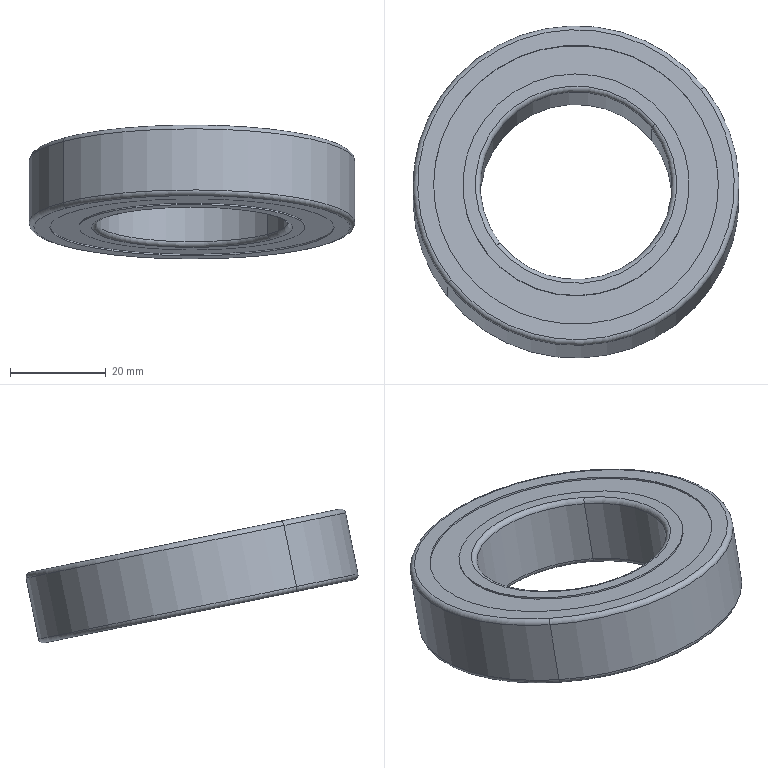Component | SolidWorks | B6008ZZ-2 | 1 solid | 26 faces | box 68 x 69.27 x 27.93 mm | volume 34781 mm3 | cylinder 12 | torus 8 | plane 6 | commonest cylinder face diameters 47.2 x4 59.4 x4 68 x2 40 x2
build123d program:
from build123d import *


with BuildPart() as part:
    # Sketch1 → Revolve1 (revolve)
    with BuildSketch(Plane.XY, mode=Mode.PRIVATE) as revolve1_sk:
        with BuildLine():
            Line((1, 20), (14, 20))
            ThreePointArc((14, 20), (14.707, 20.293), (15, 21))
            Line((15, 21), (15, 23.6))
            Line((15, 23.6), (14.658, 23.6))
            Line((14.658, 23.6), (14.658, 29.7))
            Line((14.658, 29.7), (15, 29.7))
            Line((15, 29.7), (15, 33))
            ThreePointArc((15, 33), (14.707, 33.707), (14, 34))
            Line((14, 34), (1, 34))
            ThreePointArc((1, 34), (0.2929, 33.707), (0, 33))
            Line((0, 33), (0, 29.7))
            Line((0, 29.7), (0.342, 29.7))
            Line((0.342, 29.7), (0.342, 23.6))
            Line((0.342, 23.6), (0, 23.6))
            Line((0, 23.6), (0, 21))
            ThreePointArc((0, 21), (0.2929, 20.293), (1, 20))
        make_face()
    revolve(revolve1_sk.sketch.rotate(Axis((15, 0, 0), (-1, 0, 0)), 270), axis=Axis((15, 0, 0), (-1, 0, 0)))


solid = part.part

# Placed as in the assembly
solid = solid.moved(Location((0, 169.727, 2.1), (78.465, 89.752, 90)))
STEP:
#1=CARTESIAN_POINT('',(-0.733,6.125,0.21));
#2=VERTEX_POINT('',#1);
#3=CARTESIAN_POINT('',(0.733,7.244,-0.01832));
#4=VERTEX_POINT('',#3);
#5=CARTESIAN_POINT('',(-0.,6.685,0.09585));
#6=DIRECTION('',(0.,-0.2,-0.9798));
#7=DIRECTION('',(-0.7889,-0.6021,0.1229));
#8=AXIS2_PLACEMENT_3D('',#5,#6,#7);
#9=CIRCLE('',#8,0.9291);
#10=EDGE_CURVE('',#2,#4,#9,.T.);
#11=ORIENTED_EDGE('',*,*,#10,.T.);
#12=CARTESIAN_POINT('',(0.733,7.242,-0.03152));
#13=VERTEX_POINT('',#12);
#14=CARTESIAN_POINT('',(0.733,7.36,0.5471));
#15=DIRECTION('',(0.,-0.2,-0.9798));
#16=VECTOR('',#15,39.37);
#17=LINE('',#14,#16);
#18=EDGE_CURVE('',#4,#13,#17,.T.);
#19=ORIENTED_EDGE('',*,*,#18,.T.);
#20=CARTESIAN_POINT('',(-0.733,6.123,0.1968));
#21=VERTEX_POINT('',#20);
#22=CARTESIAN_POINT('',(-0.,6.682,0.08266));
#23=DIRECTION('',(0.,-0.2,-0.9798));
#24=DIRECTION('',(-0.7889,-0.6021,0.1229));
#25=AXIS2_PLACEMENT_3D('',#22,#23,#24);
#26=CIRCLE('',#25,0.9291);
#27=EDGE_CURVE('',#21,#13,#26,.T.);
#28=ORIENTED_EDGE('',*,*,#27,.F.);
#29=CARTESIAN_POINT('',(-0.733,6.241,0.7755));
#30=DIRECTION('',(0.,-0.2,-0.9798));
#31=VECTOR('',#30,39.37);
#32=LINE('',#29,#31);
#33=EDGE_CURVE('',#2,#21,#32,.T.);
#34=ORIENTED_EDGE('',*,*,#33,.F.);
#35=EDGE_LOOP('',(#11,#19,#28,#34));
#36=FACE_OUTER_BOUND('',#35,.T.);
#37=CARTESIAN_POINT('',(-0.,6.8,0.6613));
#38=DIRECTION('',(0.,-0.2,-0.9798));
#39=DIRECTION('',(-0.7889,-0.6021,0.1229));
#40=AXIS2_PLACEMENT_3D('',#37,#38,#39);
#41=CYLINDRICAL_SURFACE('',#40,0.9291);
#42=ADVANCED_FACE('',(#36),#41,.T.);
#43=CARTESIAN_POINT('',(0.9224,7.389,-0.04784));
#44=VERTEX_POINT('',#43);
#45=CARTESIAN_POINT('',(-0.9224,5.981,0.2395));
#46=VERTEX_POINT('',#45);
#47=CARTESIAN_POINT('',(-0.,6.685,0.09585));
#48=DIRECTION('',(0.,-0.2,-0.9798));
#49=DIRECTION('',(-0.7889,-0.6021,0.1229));
#50=AXIS2_PLACEMENT_3D('',#47,#48,#49);
#51=CIRCLE('',#50,1.169);
#52=EDGE_CURVE('',#44,#46,#51,.T.);
#53=ORIENTED_EDGE('',*,*,#52,.F.);
#54=CARTESIAN_POINT('',(0.9224,7.386,-0.06103));
#55=VERTEX_POINT('',#54);
#56=CARTESIAN_POINT('',(0.9224,7.504,0.5176));
#57=DIRECTION('',(0.,-0.2,-0.9798));
#58=VECTOR('',#57,39.37);
#59=LINE('',#56,#58);
#60=EDGE_CURVE('',#44,#55,#59,.T.);
#61=ORIENTED_EDGE('',*,*,#60,.T.);
#62=CARTESIAN_POINT('',(-0.9224,5.978,0.2263));
#63=VERTEX_POINT('',#62);
#64=CARTESIAN_POINT('',(-0.,6.682,0.08266));
#65=DIRECTION('',(0.,-0.2,-0.9798));
#66=DIRECTION('',(-0.7889,-0.6021,0.1229));
#67=AXIS2_PLACEMENT_3D('',#64,#65,#66);
#68=CIRCLE('',#67,1.169);
#69=EDGE_CURVE('',#55,#63,#68,.T.);
#70=ORIENTED_EDGE('',*,*,#69,.T.);
#71=CARTESIAN_POINT('',(-0.9224,6.096,0.805));
#72=DIRECTION('',(0.,-0.2,-0.9798));
#73=VECTOR('',#72,39.37);
#74=LINE('',#71,#73);
#75=EDGE_CURVE('',#46,#63,#74,.T.);
#76=ORIENTED_EDGE('',*,*,#75,.F.);
#77=EDGE_LOOP('',(#53,#61,#70,#76));
#78=FACE_OUTER_BOUND('',#77,.T.);
#79=CARTESIAN_POINT('',(-0.,6.8,0.6613));
#80=DIRECTION('',(0.,-0.2,-0.9798));
#81=DIRECTION('',(-0.7889,-0.6021,0.1229));
#82=AXIS2_PLACEMENT_3D('',#79,#80,#81);
#83=CYLINDRICAL_SURFACE('',#82,1.169);
#84=ADVANCED_FACE('',(#78),#83,.F.);
#85=CARTESIAN_POINT('',(-1.056,5.884,0.2857));
#86=VERTEX_POINT('',#85);
#87=CARTESIAN_POINT('',(1.056,7.496,-0.04326));
#88=VERTEX_POINT('',#87);
#89=CARTESIAN_POINT('',(-0.,6.69,0.1212));
#90=DIRECTION('',(0.,-0.2,-0.9798));
#91=DIRECTION('',(-0.7889,-0.6021,0.1229));
#92=AXIS2_PLACEMENT_3D('',#89,#90,#91);
#93=CIRCLE('',#92,1.339);
#94=EDGE_CURVE('',#86,#88,#93,.T.);
#95=ORIENTED_EDGE('',*,*,#94,.T.);
#96=CARTESIAN_POINT('',(1.025,7.464,-0.07699));
#97=VERTEX_POINT('',#96);
#98=CARTESIAN_POINT('',(1.025,7.472,-0.03842));
#99=DIRECTION('',(-0.6145,0.7729,-0.1577));
#100=DIRECTION('',(-0.7827,-0.6223,0.));
#101=AXIS2_PLACEMENT_3D('',#98,#99,#100);
#102=CIRCLE('',#101,0.03937);
#103=EDGE_CURVE('',#88,#97,#102,.T.);
#104=ORIENTED_EDGE('',*,*,#103,.T.);
#105=CARTESIAN_POINT('',(-1.025,5.9,0.2423));
#106=VERTEX_POINT('',#105);
#107=CARTESIAN_POINT('',(-0.,6.682,0.08266));
#108=DIRECTION('',(0.,-0.2,-0.9798));
#109=DIRECTION('',(-0.7889,-0.6021,0.1229));
#110=AXIS2_PLACEMENT_3D('',#107,#108,#109);
#111=CIRCLE('',#110,1.299);
#112=EDGE_CURVE('',#106,#97,#111,.T.);
#113=ORIENTED_EDGE('',*,*,#112,.F.);
#114=CARTESIAN_POINT('',(-1.025,5.908,0.2809));
#115=DIRECTION('',(0.6145,-0.7729,0.1577));
#116=DIRECTION('',(0.7827,0.6223,0.));
#117=AXIS2_PLACEMENT_3D('',#114,#115,#116);
#118=CIRCLE('',#117,0.03937);
#119=EDGE_CURVE('',#86,#106,#118,.T.);
#120=ORIENTED_EDGE('',*,*,#119,.F.);
#121=EDGE_LOOP('',(#95,#104,#113,#120));
#122=FACE_OUTER_BOUND('',#121,.T.);
#123=CARTESIAN_POINT('',(-0.,6.69,0.1212));
#124=DIRECTION('',(0.,-0.2,-0.9798));
#125=DIRECTION('',(-0.7889,-0.6021,0.1229));
#126=AXIS2_PLACEMENT_3D('',#123,#124,#125);
#127=TOROIDAL_SURFACE('',#126,1.299,0.03937);
#128=ADVANCED_FACE('',(#122),#127,.T.);
#129=CARTESIAN_POINT('',(-1.056,5.986,0.7872));
#130=VERTEX_POINT('',#129);
#131=CARTESIAN_POINT('',(1.056,7.598,0.4582));
#132=VERTEX_POINT('',#131);
#133=CARTESIAN_POINT('',(-0.,6.792,0.6227));
#134=DIRECTION('',(0.,-0.2,-0.9798));
#135=DIRECTION('',(-0.7889,-0.6021,0.1229));
#136=AXIS2_PLACEMENT_3D('',#133,#134,#135);
#137=CIRCLE('',#136,1.339);
#138=EDGE_CURVE('',#130,#132,#137,.T.);
#139=ORIENTED_EDGE('',*,*,#138,.T.);
#140=CARTESIAN_POINT('',(1.056,7.606,0.4968));
#141=DIRECTION('',(0.,-0.2,-0.9798));
#142=VECTOR('',#141,39.37);
#143=LINE('',#140,#142);
#144=EDGE_CURVE('',#132,#88,#143,.T.);
#145=ORIENTED_EDGE('',*,*,#144,.T.);
#146=ORIENTED_EDGE('',*,*,#94,.F.);
#147=CARTESIAN_POINT('',(-1.056,5.994,0.8258));
#148=DIRECTION('',(0.,-0.2,-0.9798));
#149=VECTOR('',#148,39.37);
#150=LINE('',#147,#149);
#151=EDGE_CURVE('',#130,#86,#150,.T.);
#152=ORIENTED_EDGE('',*,*,#151,.F.);
#153=EDGE_LOOP('',(#139,#145,#146,#152));
#154=FACE_OUTER_BOUND('',#153,.T.);
#155=CARTESIAN_POINT('',(-0.,6.8,0.6613));
#156=DIRECTION('',(0.,-0.2,-0.9798));
#157=DIRECTION('',(-0.7889,-0.6021,0.1229));
#158=AXIS2_PLACEMENT_3D('',#155,#156,#157);
#159=CYLINDRICAL_SURFACE('',#158,1.339);
#160=ADVANCED_FACE('',(#154),#159,.T.);
#161=CARTESIAN_POINT('',(-1.025,6.018,0.8209));
#162=VERTEX_POINT('',#161);
#163=CARTESIAN_POINT('',(1.025,7.583,0.5016));
#164=VERTEX_POINT('',#163);
#165=CARTESIAN_POINT('',(-0.,6.8,0.6613));
#166=DIRECTION('',(0.,-0.2,-0.9798));
#167=DIRECTION('',(-0.7889,-0.6021,0.1229));
#168=AXIS2_PLACEMENT_3D('',#165,#166,#167);
#169=CIRCLE('',#168,1.299);
#170=EDGE_CURVE('',#162,#164,#169,.T.);
#171=ORIENTED_EDGE('',*,*,#170,.T.);
#172=CARTESIAN_POINT('',(1.025,7.575,0.4631));
#173=DIRECTION('',(-0.6145,0.7729,-0.1577));
#174=DIRECTION('',(-0.7827,-0.6223,0.));
#175=AXIS2_PLACEMENT_3D('',#172,#173,#174);
#176=CIRCLE('',#175,0.03937);
#177=EDGE_CURVE('',#164,#132,#176,.T.);
#178=ORIENTED_EDGE('',*,*,#177,.T.);
#179=ORIENTED_EDGE('',*,*,#138,.F.);
#180=CARTESIAN_POINT('',(-1.025,6.01,0.7824));
#181=DIRECTION('',(0.6145,-0.7729,0.1577));
#182=DIRECTION('',(0.7827,0.6223,0.));
#183=AXIS2_PLACEMENT_3D('',#180,#181,#182);
#184=CIRCLE('',#183,0.03937);
#185=EDGE_CURVE('',#162,#130,#184,.T.);
#186=ORIENTED_EDGE('',*,*,#185,.F.);
#187=EDGE_LOOP('',(#171,#178,#179,#186));
#188=FACE_OUTER_BOUND('',#187,.T.);
#189=CARTESIAN_POINT('',(-0.,6.792,0.6227));
#190=DIRECTION('',(0.,-0.2,-0.9798));
#191=DIRECTION('',(-0.7889,-0.6021,0.1229));
#192=AXIS2_PLACEMENT_3D('',#189,#190,#191);
#193=TOROIDAL_SURFACE('',#192,1.299,0.03937);
#194=ADVANCED_FACE('',(#188),#193,.T.);
#195=CARTESIAN_POINT('',(0.9224,7.504,0.5176));
#196=VERTEX_POINT('',#195);
#197=CARTESIAN_POINT('',(-0.9224,6.096,0.805));
#198=VERTEX_POINT('',#197);
#199=CARTESIAN_POINT('',(-0.,6.8,0.6613));
#200=DIRECTION('',(0.,-0.2,-0.9798));
#201=DIRECTION('',(-0.7889,-0.6021,0.1229));
#202=AXIS2_PLACEMENT_3D('',#199,#200,#201);
#203=CIRCLE('',#202,1.169);
#204=EDGE_CURVE('',#196,#198,#203,.T.);
#205=ORIENTED_EDGE('',*,*,#204,.F.);
#206=CARTESIAN_POINT('',(0.9224,7.502,0.5044));
#207=VERTEX_POINT('',#206);
#208=CARTESIAN_POINT('',(0.9224,7.504,0.5176));
#209=DIRECTION('',(0.,-0.2,-0.9798));
#210=VECTOR('',#209,39.37);
#211=LINE('',#208,#210);
#212=EDGE_CURVE('',#196,#207,#211,.T.);
#213=ORIENTED_EDGE('',*,*,#212,.T.);
#214=CARTESIAN_POINT('',(-0.9224,6.093,0.7918));
#215=VERTEX_POINT('',#214);
#216=CARTESIAN_POINT('',(-0.,6.798,0.6481));
#217=DIRECTION('',(0.,-0.2,-0.9798));
#218=DIRECTION('',(-0.7889,-0.6021,0.1229));
#219=AXIS2_PLACEMENT_3D('',#216,#217,#218);
#220=CIRCLE('',#219,1.169);
#221=EDGE_CURVE('',#207,#215,#220,.T.);
#222=ORIENTED_EDGE('',*,*,#221,.T.);
#223=CARTESIAN_POINT('',(-0.9224,6.096,0.805));
#224=DIRECTION('',(0.,-0.2,-0.9798));
#225=VECTOR('',#224,39.37);
#226=LINE('',#223,#225);
#227=EDGE_CURVE('',#198,#215,#226,.T.);
#228=ORIENTED_EDGE('',*,*,#227,.F.);
#229=EDGE_LOOP('',(#205,#213,#222,#228));
#230=FACE_OUTER_BOUND('',#229,.T.);
#231=CARTESIAN_POINT('',(-0.,6.8,0.6613));
#232=DIRECTION('',(0.,-0.2,-0.9798));
#233=DIRECTION('',(-0.7889,-0.6021,0.1229));
#234=AXIS2_PLACEMENT_3D('',#231,#232,#233);
#235=CYLINDRICAL_SURFACE('',#234,1.169);
#236=ADVANCED_FACE('',(#230),#235,.F.);
#237=CARTESIAN_POINT('',(-0.733,6.241,0.7755));
#238=VERTEX_POINT('',#237);
#239=CARTESIAN_POINT('',(0.733,7.36,0.5471));
#240=VERTEX_POINT('',#239);
#241=CARTESIAN_POINT('',(-0.,6.8,0.6613));
#242=DIRECTION('',(0.,-0.2,-0.9798));
#243=DIRECTION('',(-0.7889,-0.6021,0.1229));
#244=AXIS2_PLACEMENT_3D('',#241,#242,#243);
#245=CIRCLE('',#244,0.9291);
#246=EDGE_CURVE('',#238,#240,#245,.T.);
#247=ORIENTED_EDGE('',*,*,#246,.T.);
#248=CARTESIAN_POINT('',(0.733,7.357,0.5339));
#249=VERTEX_POINT('',#248);
#250=CARTESIAN_POINT('',(0.733,7.36,0.5471));
#251=DIRECTION('',(0.,-0.2,-0.9798));
#252=VECTOR('',#251,39.37);
#253=LINE('',#250,#252);
#254=EDGE_CURVE('',#240,#249,#253,.T.);
#255=ORIENTED_EDGE('',*,*,#254,.T.);
#256=CARTESIAN_POINT('',(-0.733,6.238,0.7623));
#257=VERTEX_POINT('',#256);
#258=CARTESIAN_POINT('',(-0.,6.798,0.6481));
#259=DIRECTION('',(0.,-0.2,-0.9798));
#260=DIRECTION('',(-0.7889,-0.6021,0.1229));
#261=AXIS2_PLACEMENT_3D('',#258,#259,#260);
#262=CIRCLE('',#261,0.9291);
#263=EDGE_CURVE('',#257,#249,#262,.T.);
#264=ORIENTED_EDGE('',*,*,#263,.F.);
#265=CARTESIAN_POINT('',(-0.733,6.241,0.7755));
#266=DIRECTION('',(0.,-0.2,-0.9798));
#267=VECTOR('',#266,39.37);
#268=LINE('',#265,#267);
#269=EDGE_CURVE('',#238,#257,#268,.T.);
#270=ORIENTED_EDGE('',*,*,#269,.F.);
#271=EDGE_LOOP('',(#247,#255,#264,#270));
#272=FACE_OUTER_BOUND('',#271,.T.);
#273=CARTESIAN_POINT('',(-0.,6.8,0.6613));
#274=DIRECTION('',(0.,-0.2,-0.9798));
#275=DIRECTION('',(-0.7889,-0.6021,0.1229));
#276=AXIS2_PLACEMENT_3D('',#273,#274,#275);
#277=CYLINDRICAL_SURFACE('',#276,0.9291);
#278=ADVANCED_FACE('',(#272),#277,.T.);
#279=CARTESIAN_POINT('',(-0.6212,6.318,0.7195));
#280=VERTEX_POINT('',#279);
#281=CARTESIAN_POINT('',(0.6212,7.267,0.526));
#282=VERTEX_POINT('',#281);
#283=CARTESIAN_POINT('',(-0.,6.792,0.6227));
#284=DIRECTION('',(0.,-0.2,-0.9798));
#285=DIRECTION('',(-0.7889,-0.6021,0.1229));
#286=AXIS2_PLACEMENT_3D('',#283,#284,#285);
#287=CIRCLE('',#286,0.7874);
#288=EDGE_CURVE('',#280,#282,#287,.T.);
#289=ORIENTED_EDGE('',*,*,#288,.T.);
#290=CARTESIAN_POINT('',(0.6522,7.298,0.5597));
#291=VERTEX_POINT('',#290);
#292=CARTESIAN_POINT('',(0.6522,7.29,0.5211));
#293=DIRECTION('',(-0.6145,0.7729,-0.1577));
#294=DIRECTION('',(-0.7827,-0.6223,0.));
#295=AXIS2_PLACEMENT_3D('',#292,#293,#294);
#296=CIRCLE('',#295,0.03937);
#297=EDGE_CURVE('',#282,#291,#296,.T.);
#298=ORIENTED_EDGE('',*,*,#297,.T.);
#299=CARTESIAN_POINT('',(-0.6522,6.302,0.7629));
#300=VERTEX_POINT('',#299);
#301=CARTESIAN_POINT('',(-0.,6.8,0.6613));
#302=DIRECTION('',(0.,-0.2,-0.9798));
#303=DIRECTION('',(-0.7889,-0.6021,0.1229));
#304=AXIS2_PLACEMENT_3D('',#301,#302,#303);
#305=CIRCLE('',#304,0.8268);
#306=EDGE_CURVE('',#300,#291,#305,.T.);
#307=ORIENTED_EDGE('',*,*,#306,.F.);
#308=CARTESIAN_POINT('',(-0.6522,6.295,0.7243));
#309=DIRECTION('',(0.6145,-0.7729,0.1577));
#310=DIRECTION('',(0.7827,0.6223,0.));
#311=AXIS2_PLACEMENT_3D('',#308,#309,#310);
#312=CIRCLE('',#311,0.03937);
#313=EDGE_CURVE('',#280,#300,#312,.T.);
#314=ORIENTED_EDGE('',*,*,#313,.F.);
#315=EDGE_LOOP('',(#289,#298,#307,#314));
#316=FACE_OUTER_BOUND('',#315,.T.);
#317=CARTESIAN_POINT('',(-0.,6.792,0.6227));
#318=DIRECTION('',(0.,-0.2,-0.9798));
#319=DIRECTION('',(-0.7889,-0.6021,0.1229));
#320=AXIS2_PLACEMENT_3D('',#317,#318,#319);
#321=TOROIDAL_SURFACE('',#320,0.8268,0.03937);
#322=ADVANCED_FACE('',(#316),#321,.T.);
#323=CARTESIAN_POINT('',(-0.,6.792,0.6227));
#324=DIRECTION('',(0.,-0.2,-0.9798));
#325=DIRECTION('',(-0.7889,-0.6021,0.1229));
#326=AXIS2_PLACEMENT_3D('',#323,#324,#325);
#327=CIRCLE('',#326,0.7874);
#328=EDGE_CURVE('',#282,#280,#327,.T.);
#329=ORIENTED_EDGE('',*,*,#328,.F.);
#330=CARTESIAN_POINT('',(0.6212,7.164,0.02448));
#331=VERTEX_POINT('',#330);
#332=CARTESIAN_POINT('',(0.6212,7.274,0.5645));
#333=DIRECTION('',(0.,-0.2,-0.9798));
#334=VECTOR('',#333,39.37);
#335=LINE('',#332,#334);
#336=EDGE_CURVE('',#282,#331,#335,.T.);
#337=ORIENTED_EDGE('',*,*,#336,.T.);
#338=CARTESIAN_POINT('',(-0.6212,6.216,0.218));
#339=VERTEX_POINT('',#338);
#340=CARTESIAN_POINT('',(-0.,6.69,0.1212));
#341=DIRECTION('',(0.,-0.2,-0.9798));
#342=DIRECTION('',(-0.7889,-0.6021,0.1229));
#343=AXIS2_PLACEMENT_3D('',#340,#341,#342);
#344=CIRCLE('',#343,0.7874);
#345=EDGE_CURVE('',#331,#339,#344,.T.);
#346=ORIENTED_EDGE('',*,*,#345,.T.);
#347=CARTESIAN_POINT('',(-0.6212,6.326,0.758));
#348=DIRECTION('',(0.,-0.2,-0.9798));
#349=VECTOR('',#348,39.37);
#350=LINE('',#347,#349);
#351=EDGE_CURVE('',#280,#339,#350,.T.);
#352=ORIENTED_EDGE('',*,*,#351,.F.);
#353=EDGE_LOOP('',(#329,#337,#346,#352));
#354=FACE_OUTER_BOUND('',#353,.T.);
#355=CARTESIAN_POINT('',(-0.,6.8,0.6613));
#356=DIRECTION('',(0.,-0.2,-0.9798));
#357=DIRECTION('',(-0.7889,-0.6021,0.1229));
#358=AXIS2_PLACEMENT_3D('',#355,#356,#357);
#359=CYLINDRICAL_SURFACE('',#358,0.7874);
#360=ADVANCED_FACE('',(#354),#359,.F.);
#361=CARTESIAN_POINT('',(-0.6522,6.184,0.1843));
#362=VERTEX_POINT('',#361);
#363=CARTESIAN_POINT('',(0.6522,7.18,-0.01894));
#364=VERTEX_POINT('',#363);
#365=CARTESIAN_POINT('',(-0.,6.682,0.08266));
#366=DIRECTION('',(0.,-0.2,-0.9798));
#367=DIRECTION('',(-0.7889,-0.6021,0.1229));
#368=AXIS2_PLACEMENT_3D('',#365,#366,#367);
#369=CIRCLE('',#368,0.8268);
#370=EDGE_CURVE('',#362,#364,#369,.T.);
#371=ORIENTED_EDGE('',*,*,#370,.T.);
#372=CARTESIAN_POINT('',(0.6522,7.188,0.01964));
#373=DIRECTION('',(-0.6145,0.7729,-0.1577));
#374=DIRECTION('',(-0.7827,-0.6223,0.));
#375=AXIS2_PLACEMENT_3D('',#372,#373,#374);
#376=CIRCLE('',#375,0.03937);
#377=EDGE_CURVE('',#364,#331,#376,.T.);
#378=ORIENTED_EDGE('',*,*,#377,.T.);
#379=CARTESIAN_POINT('',(-0.,6.69,0.1212));
#380=DIRECTION('',(0.,-0.2,-0.9798));
#381=DIRECTION('',(-0.7889,-0.6021,0.1229));
#382=AXIS2_PLACEMENT_3D('',#379,#380,#381);
#383=CIRCLE('',#382,0.7874);
#384=EDGE_CURVE('',#339,#331,#383,.T.);
#385=ORIENTED_EDGE('',*,*,#384,.F.);
#386=CARTESIAN_POINT('',(-0.6522,6.192,0.2228));
#387=DIRECTION('',(0.6145,-0.7729,0.1577));
#388=DIRECTION('',(0.7827,0.6223,0.));
#389=AXIS2_PLACEMENT_3D('',#386,#387,#388);
#390=CIRCLE('',#389,0.03937);
#391=EDGE_CURVE('',#362,#339,#390,.T.);
#392=ORIENTED_EDGE('',*,*,#391,.F.);
#393=EDGE_LOOP('',(#371,#378,#385,#392));
#394=FACE_OUTER_BOUND('',#393,.T.);
#395=CARTESIAN_POINT('',(-0.,6.69,0.1212));
#396=DIRECTION('',(0.,-0.2,-0.9798));
#397=DIRECTION('',(-0.7889,-0.6021,0.1229));
#398=AXIS2_PLACEMENT_3D('',#395,#396,#397);
#399=TOROIDAL_SURFACE('',#398,0.8268,0.03937);
#400=ADVANCED_FACE('',(#394),#399,.T.);
#401=ORIENTED_EDGE('',*,*,#377,.F.);
#402=CARTESIAN_POINT('',(-0.,6.682,0.08266));
#403=DIRECTION('',(0.,-0.2,-0.9798));
#404=DIRECTION('',(-0.7889,-0.6021,0.1229));
#405=AXIS2_PLACEMENT_3D('',#402,#403,#404);
#406=CIRCLE('',#405,0.8268);
#407=EDGE_CURVE('',#364,#362,#406,.T.);
#408=ORIENTED_EDGE('',*,*,#407,.T.);
#409=ORIENTED_EDGE('',*,*,#391,.T.);
#410=ORIENTED_EDGE('',*,*,#345,.F.);
#411=EDGE_LOOP('',(#401,#408,#409,#410));
#412=FACE_OUTER_BOUND('',#411,.T.);
#413=CARTESIAN_POINT('',(-0.,6.69,0.1212));
#414=DIRECTION('',(0.,-0.2,-0.9798));
#415=DIRECTION('',(-0.7889,-0.6021,0.1229));
#416=AXIS2_PLACEMENT_3D('',#413,#414,#415);
#417=TOROIDAL_SURFACE('',#416,0.8268,0.03937);
#418=ADVANCED_FACE('',(#412),#417,.T.);
#419=ORIENTED_EDGE('',*,*,#336,.F.);
#420=ORIENTED_EDGE('',*,*,#288,.F.);
#421=ORIENTED_EDGE('',*,*,#351,.T.);
#422=ORIENTED_EDGE('',*,*,#384,.T.);
#423=EDGE_LOOP('',(#419,#420,#421,#422));
#424=FACE_OUTER_BOUND('',#423,.T.);
#425=CARTESIAN_POINT('',(-0.,6.8,0.6613));
#426=DIRECTION('',(0.,-0.2,-0.9798));
#427=DIRECTION('',(-0.7889,-0.6021,0.1229));
#428=AXIS2_PLACEMENT_3D('',#425,#426,#427);
#429=CYLINDRICAL_SURFACE('',#428,0.7874);
#430=ADVANCED_FACE('',(#424),#429,.F.);
#431=ORIENTED_EDGE('',*,*,#297,.F.);
#432=ORIENTED_EDGE('',*,*,#328,.T.);
#433=ORIENTED_EDGE('',*,*,#313,.T.);
#434=CARTESIAN_POINT('',(-0.,6.8,0.6613));
#435=DIRECTION('',(0.,-0.2,-0.9798));
#436=DIRECTION('',(-0.7889,-0.6021,0.1229));
#437=AXIS2_PLACEMENT_3D('',#434,#435,#436);
#438=CIRCLE('',#437,0.8268);
#439=EDGE_CURVE('',#291,#300,#438,.T.);
#440=ORIENTED_EDGE('',*,*,#439,.F.);
#441=EDGE_LOOP('',(#431,#432,#433,#440));
#442=FACE_OUTER_BOUND('',#441,.T.);
#443=CARTESIAN_POINT('',(-0.,6.792,0.6227));
#444=DIRECTION('',(0.,-0.2,-0.9798));
#445=DIRECTION('',(-0.7889,-0.6021,0.1229));
#446=AXIS2_PLACEMENT_3D('',#443,#444,#445);
#447=TOROIDAL_SURFACE('',#446,0.8268,0.03937);
#448=ADVANCED_FACE('',(#442),#447,.T.);
#449=ORIENTED_EDGE('',*,*,#246,.F.);
#450=CARTESIAN_POINT('',(-0.,6.8,0.6613));
#451=DIRECTION('',(0.,-0.2,-0.9798));
#452=DIRECTION('',(-0.7889,-0.6021,0.1229));
#453=AXIS2_PLACEMENT_3D('',#450,#451,#452);
#454=CIRCLE('',#453,0.9291);
#455=EDGE_CURVE('',#240,#238,#454,.T.);
#456=ORIENTED_EDGE('',*,*,#455,.F.);
#457=EDGE_LOOP('',(#449,#456));
#458=FACE_OUTER_BOUND('',#457,.T.);
#459=ORIENTED_EDGE('',*,*,#306,.T.);
#460=ORIENTED_EDGE('',*,*,#439,.T.);
#461=EDGE_LOOP('',(#459,#460));
#462=FACE_BOUND('',#461,.T.);
#463=CARTESIAN_POINT('',(-0.5081,7.439,0.5309));
#464=DIRECTION('',(0.,-0.2,-0.9798));
#465=DIRECTION('',(-0.7889,-0.6021,0.1229));
#466=AXIS2_PLACEMENT_3D('',#463,#464,#465);
#467=PLANE('',#466);
#468=ADVANCED_FACE('',(#458,#462),#467,.F.);
#469=ORIENTED_EDGE('',*,*,#254,.F.);
#470=ORIENTED_EDGE('',*,*,#455,.T.);
#471=ORIENTED_EDGE('',*,*,#269,.T.);
#472=CARTESIAN_POINT('',(-0.,6.798,0.6481));
#473=DIRECTION('',(0.,-0.2,-0.9798));
#474=DIRECTION('',(-0.7889,-0.6021,0.1229));
#475=AXIS2_PLACEMENT_3D('',#472,#473,#474);
#476=CIRCLE('',#475,0.9291);
#477=EDGE_CURVE('',#249,#257,#476,.T.);
#478=ORIENTED_EDGE('',*,*,#477,.F.);
#479=EDGE_LOOP('',(#469,#470,#471,#478));
#480=FACE_OUTER_BOUND('',#479,.T.);
#481=CARTESIAN_POINT('',(-0.,6.8,0.6613));
#482=DIRECTION('',(0.,-0.2,-0.9798));
#483=DIRECTION('',(-0.7889,-0.6021,0.1229));
#484=AXIS2_PLACEMENT_3D('',#481,#482,#483);
#485=CYLINDRICAL_SURFACE('',#484,0.9291);
#486=ADVANCED_FACE('',(#480),#485,.T.);
#487=CARTESIAN_POINT('',(-0.,6.798,0.6481));
#488=DIRECTION('',(0.,-0.2,-0.9798));
#489=DIRECTION('',(-0.7889,-0.6021,0.1229));
#490=AXIS2_PLACEMENT_3D('',#487,#488,#489);
#491=CIRCLE('',#490,1.169);
#492=EDGE_CURVE('',#215,#207,#491,.T.);
#493=ORIENTED_EDGE('',*,*,#492,.F.);
#494=ORIENTED_EDGE('',*,*,#221,.F.);
#495=EDGE_LOOP('',(#493,#494));
#496=FACE_OUTER_BOUND('',#495,.T.);
#497=ORIENTED_EDGE('',*,*,#263,.T.);
#498=ORIENTED_EDGE('',*,*,#477,.T.);
#499=EDGE_LOOP('',(#497,#498));
#500=FACE_BOUND('',#499,.T.);
#501=CARTESIAN_POINT('',(-0.571,7.516,0.5015));
#502=DIRECTION('',(0.,-0.2,-0.9798));
#503=DIRECTION('',(-0.7889,-0.6021,0.1229));
#504=AXIS2_PLACEMENT_3D('',#501,#502,#503);
#505=PLANE('',#504);
#506=ADVANCED_FACE('',(#496,#500),#505,.F.);
#507=ORIENTED_EDGE('',*,*,#212,.F.);
#508=CARTESIAN_POINT('',(-0.,6.8,0.6613));
#509=DIRECTION('',(0.,-0.2,-0.9798));
#510=DIRECTION('',(-0.7889,-0.6021,0.1229));
#511=AXIS2_PLACEMENT_3D('',#508,#509,#510);
#512=CIRCLE('',#511,1.169);
#513=EDGE_CURVE('',#198,#196,#512,.T.);
#514=ORIENTED_EDGE('',*,*,#513,.F.);
#515=ORIENTED_EDGE('',*,*,#227,.T.);
#516=ORIENTED_EDGE('',*,*,#492,.T.);
#517=EDGE_LOOP('',(#507,#514,#515,#516));
#518=FACE_OUTER_BOUND('',#517,.T.);
#519=CARTESIAN_POINT('',(-0.,6.8,0.6613));
#520=DIRECTION('',(0.,-0.2,-0.9798));
#521=DIRECTION('',(-0.7889,-0.6021,0.1229));
#522=AXIS2_PLACEMENT_3D('',#519,#520,#521);
#523=CYLINDRICAL_SURFACE('',#522,1.169);
#524=ADVANCED_FACE('',(#518),#523,.F.);
#525=ORIENTED_EDGE('',*,*,#170,.F.);
#526=CARTESIAN_POINT('',(-0.,6.8,0.6613));
#527=DIRECTION('',(0.,-0.2,-0.9798));
#528=DIRECTION('',(-0.7889,-0.6021,0.1229));
#529=AXIS2_PLACEMENT_3D('',#526,#527,#528);
#530=CIRCLE('',#529,1.299);
#531=EDGE_CURVE('',#164,#162,#530,.T.);
#532=ORIENTED_EDGE('',*,*,#531,.F.);
#533=EDGE_LOOP('',(#525,#532));
#534=FACE_OUTER_BOUND('',#533,.T.);
#535=ORIENTED_EDGE('',*,*,#513,.T.);
#536=ORIENTED_EDGE('',*,*,#204,.T.);
#537=EDGE_LOOP('',(#535,#536));
#538=FACE_BOUND('',#537,.T.);
#539=CARTESIAN_POINT('',(-0.7186,7.704,0.4768));
#540=DIRECTION('',(0.,-0.2,-0.9798));
#541=DIRECTION('',(-0.7889,-0.6021,0.1229));
#542=AXIS2_PLACEMENT_3D('',#539,#540,#541);
#543=PLANE('',#542);
#544=ADVANCED_FACE('',(#534,#538),#543,.F.);
#545=ORIENTED_EDGE('',*,*,#177,.F.);
#546=ORIENTED_EDGE('',*,*,#531,.T.);
#547=ORIENTED_EDGE('',*,*,#185,.T.);
#548=CARTESIAN_POINT('',(-0.,6.792,0.6227));
#549=DIRECTION('',(0.,-0.2,-0.9798));
#550=DIRECTION('',(-0.7889,-0.6021,0.1229));
#551=AXIS2_PLACEMENT_3D('',#548,#549,#550);
#552=CIRCLE('',#551,1.339);
#553=EDGE_CURVE('',#132,#130,#552,.T.);
#554=ORIENTED_EDGE('',*,*,#553,.F.);
#555=EDGE_LOOP('',(#545,#546,#547,#554));
#556=FACE_OUTER_BOUND('',#555,.T.);
#557=CARTESIAN_POINT('',(-0.,6.792,0.6227));
#558=DIRECTION('',(0.,-0.2,-0.9798));
#559=DIRECTION('',(-0.7889,-0.6021,0.1229));
#560=AXIS2_PLACEMENT_3D('',#557,#558,#559);
#561=TOROIDAL_SURFACE('',#560,1.299,0.03937);
#562=ADVANCED_FACE('',(#556),#561,.T.);
#563=ORIENTED_EDGE('',*,*,#144,.F.);
#564=ORIENTED_EDGE('',*,*,#553,.T.);
#565=ORIENTED_EDGE('',*,*,#151,.T.);
#566=CARTESIAN_POINT('',(-0.,6.69,0.1212));
#567=DIRECTION('',(0.,-0.2,-0.9798));
#568=DIRECTION('',(-0.7889,-0.6021,0.1229));
#569=AXIS2_PLACEMENT_3D('',#566,#567,#568);
#570=CIRCLE('',#569,1.339);
#571=EDGE_CURVE('',#88,#86,#570,.T.);
#572=ORIENTED_EDGE('',*,*,#571,.F.);
#573=EDGE_LOOP('',(#563,#564,#565,#572));
#574=FACE_OUTER_BOUND('',#573,.T.);
#575=CARTESIAN_POINT('',(-0.,6.8,0.6613));
#576=DIRECTION('',(0.,-0.2,-0.9798));
#577=DIRECTION('',(-0.7889,-0.6021,0.1229));
#578=AXIS2_PLACEMENT_3D('',#575,#576,#577);
#579=CYLINDRICAL_SURFACE('',#578,1.339);
#580=ADVANCED_FACE('',(#574),#579,.T.);
#581=ORIENTED_EDGE('',*,*,#103,.F.);
#582=ORIENTED_EDGE('',*,*,#571,.T.);
#583=ORIENTED_EDGE('',*,*,#119,.T.);
#584=CARTESIAN_POINT('',(-0.,6.682,0.08266));
#585=DIRECTION('',(0.,-0.2,-0.9798));
#586=DIRECTION('',(-0.7889,-0.6021,0.1229));
#587=AXIS2_PLACEMENT_3D('',#584,#585,#586);
#588=CIRCLE('',#587,1.299);
#589=EDGE_CURVE('',#97,#106,#588,.T.);
#590=ORIENTED_EDGE('',*,*,#589,.F.);
#591=EDGE_LOOP('',(#581,#582,#583,#590));
#592=FACE_OUTER_BOUND('',#591,.T.);
#593=CARTESIAN_POINT('',(-0.,6.69,0.1212));
#594=DIRECTION('',(0.,-0.2,-0.9798));
#595=DIRECTION('',(-0.7889,-0.6021,0.1229));
#596=AXIS2_PLACEMENT_3D('',#593,#594,#595);
#597=TOROIDAL_SURFACE('',#596,1.299,0.03937);
#598=ADVANCED_FACE('',(#592),#597,.T.);
#599=CARTESIAN_POINT('',(-0.,6.682,0.08266));
#600=DIRECTION('',(0.,-0.2,-0.9798));
#601=DIRECTION('',(-0.7889,-0.6021,0.1229));
#602=AXIS2_PLACEMENT_3D('',#599,#600,#601);
#603=CIRCLE('',#602,1.169);
#604=EDGE_CURVE('',#63,#55,#603,.T.);
#605=ORIENTED_EDGE('',*,*,#604,.F.);
#606=ORIENTED_EDGE('',*,*,#69,.F.);
#607=EDGE_LOOP('',(#605,#606));
#608=FACE_BOUND('',#607,.T.);
#609=ORIENTED_EDGE('',*,*,#112,.T.);
#610=ORIENTED_EDGE('',*,*,#589,.T.);
#611=EDGE_LOOP('',(#609,#610));
#612=FACE_OUTER_BOUND('',#611,.T.);
#613=CARTESIAN_POINT('',(-0.7984,7.686,-0.1223));
#614=DIRECTION('',(-0.,0.2,0.9798));
#615=DIRECTION('',(0.7889,0.6021,-0.1229));
#616=AXIS2_PLACEMENT_3D('',#613,#614,#615);
#617=PLANE('',#616);
#618=ADVANCED_FACE('',(#608,#612),#617,.F.);
#619=ORIENTED_EDGE('',*,*,#60,.F.);
#620=CARTESIAN_POINT('',(-0.,6.685,0.09585));
#621=DIRECTION('',(0.,-0.2,-0.9798));
#622=DIRECTION('',(-0.7889,-0.6021,0.1229));
#623=AXIS2_PLACEMENT_3D('',#620,#621,#622);
#624=CIRCLE('',#623,1.169);
#625=EDGE_CURVE('',#46,#44,#624,.T.);
#626=ORIENTED_EDGE('',*,*,#625,.F.);
#627=ORIENTED_EDGE('',*,*,#75,.T.);
#628=ORIENTED_EDGE('',*,*,#604,.T.);
#629=EDGE_LOOP('',(#619,#626,#627,#628));
#630=FACE_OUTER_BOUND('',#629,.T.);
#631=CARTESIAN_POINT('',(-0.,6.8,0.6613));
#632=DIRECTION('',(0.,-0.2,-0.9798));
#633=DIRECTION('',(-0.7889,-0.6021,0.1229));
#634=AXIS2_PLACEMENT_3D('',#631,#632,#633);
#635=CYLINDRICAL_SURFACE('',#634,1.169);
#636=ADVANCED_FACE('',(#630),#635,.F.);
#637=ORIENTED_EDGE('',*,*,#10,.F.);
#638=CARTESIAN_POINT('',(-0.,6.685,0.09585));
#639=DIRECTION('',(0.,-0.2,-0.9798));
#640=DIRECTION('',(-0.7889,-0.6021,0.1229));
#641=AXIS2_PLACEMENT_3D('',#638,#639,#640);
#642=CIRCLE('',#641,0.9291);
#643=EDGE_CURVE('',#4,#2,#642,.T.);
#644=ORIENTED_EDGE('',*,*,#643,.F.);
#645=EDGE_LOOP('',(#637,#644));
#646=FACE_BOUND('',#645,.T.);
#647=ORIENTED_EDGE('',*,*,#625,.T.);
#648=ORIENTED_EDGE('',*,*,#52,.T.);
#649=EDGE_LOOP('',(#647,#648));
#650=FACE_OUTER_BOUND('',#649,.T.);
#651=CARTESIAN_POINT('',(-0.7186,7.589,-0.0886));
#652=DIRECTION('',(-0.,0.2,0.9798));
#653=DIRECTION('',(0.7889,0.6021,-0.1229));
#654=AXIS2_PLACEMENT_3D('',#651,#652,#653);
#655=PLANE('',#654);
#656=ADVANCED_FACE('',(#646,#650),#655,.F.);
#657=ORIENTED_EDGE('',*,*,#18,.F.);
#658=ORIENTED_EDGE('',*,*,#643,.T.);
#659=ORIENTED_EDGE('',*,*,#33,.T.);
#660=CARTESIAN_POINT('',(-0.,6.682,0.08266));
#661=DIRECTION('',(0.,-0.2,-0.9798));
#662=DIRECTION('',(-0.7889,-0.6021,0.1229));
#663=AXIS2_PLACEMENT_3D('',#660,#661,#662);
#664=CIRCLE('',#663,0.9291);
#665=EDGE_CURVE('',#13,#21,#664,.T.);
#666=ORIENTED_EDGE('',*,*,#665,.F.);
#667=EDGE_LOOP('',(#657,#658,#659,#666));
#668=FACE_OUTER_BOUND('',#667,.T.);
#669=CARTESIAN_POINT('',(-0.,6.8,0.6613));
#670=DIRECTION('',(0.,-0.2,-0.9798));
#671=DIRECTION('',(-0.7889,-0.6021,0.1229));
#672=AXIS2_PLACEMENT_3D('',#669,#670,#671);
#673=CYLINDRICAL_SURFACE('',#672,0.9291);
#674=ADVANCED_FACE('',(#668),#673,.T.);
#675=ORIENTED_EDGE('',*,*,#370,.F.);
#676=ORIENTED_EDGE('',*,*,#407,.F.);
#677=EDGE_LOOP('',(#675,#676));
#678=FACE_BOUND('',#677,.T.);
#679=ORIENTED_EDGE('',*,*,#27,.T.);
#680=ORIENTED_EDGE('',*,*,#665,.T.);
#681=EDGE_LOOP('',(#679,#680));
#682=FACE_OUTER_BOUND('',#681,.T.);
#683=CARTESIAN_POINT('',(-0.571,7.4,-0.0639));
#684=DIRECTION('',(-0.,0.2,0.9798));
#685=DIRECTION('',(0.7889,0.6021,-0.1229));
#686=AXIS2_PLACEMENT_3D('',#683,#684,#685);
#687=PLANE('',#686);
#688=ADVANCED_FACE('',(#678,#682),#687,.F.);
#689=CLOSED_SHELL('',(#42,#84,#128,#160,#194,#236,#278,#322,#360,#400,#418,#430,#448,#468,#486,#506,#524,#544,#562,#580,#598,#618,#636,#656,#674,#688));
#690=MANIFOLD_SOLID_BREP('',#689);
#691=CARTESIAN_POINT('',(0.,0.,0.));
#692=DIRECTION('',(0.,0.,1.));
#693=DIRECTION('',(1.,0.,0.));
#694=AXIS2_PLACEMENT_3D('',#691,#692,#693);
#695=(LENGTH_UNIT()NAMED_UNIT(*)SI_UNIT($,.METRE.));
#696=LENGTH_MEASURE_WITH_UNIT(LENGTH_MEASURE(0.0254),#695);
#697=DIMENSIONAL_EXPONENTS(1.,0.,0.,0.,0.,0.,0.);
#698=(CONVERSION_BASED_UNIT('',#696)LENGTH_UNIT()NAMED_UNIT(#697));
#699=UNCERTAINTY_MEASURE_WITH_UNIT(LENGTH_MEASURE(0.00001),#698,'','');
#700=(NAMED_UNIT(*)PLANE_ANGLE_UNIT()SI_UNIT($,.RADIAN.));
#701=(NAMED_UNIT(*)SI_UNIT($,.STERADIAN.)SOLID_ANGLE_UNIT());
#702=(GEOMETRIC_REPRESENTATION_CONTEXT(3)GLOBAL_UNCERTAINTY_ASSIGNED_CONTEXT((#699))GLOBAL_UNIT_ASSIGNED_CONTEXT((#698,#700,#701))REPRESENTATION_CONTEXT('',''));
#703=ADVANCED_BREP_SHAPE_REPRESENTATION('',(#690,#694),#702);
#704=COLOUR_RGB('',0.7922,0.8196,0.9333);
#705=FILL_AREA_STYLE_COLOUR('',#704);
#706=FILL_AREA_STYLE('',(#705));
#707=SURFACE_STYLE_FILL_AREA(#706);
#708=SURFACE_SIDE_STYLE('',(#707));
#709=SURFACE_STYLE_USAGE(.BOTH.,#708);
#710=PRESENTATION_STYLE_ASSIGNMENT((#709));
#711=STYLED_ITEM('',(#710),#690);
#712=(LENGTH_UNIT()NAMED_UNIT(*)SI_UNIT($,.METRE.));
#713=LENGTH_MEASURE_WITH_UNIT(LENGTH_MEASURE(0.0254),#712);
#714=DIMENSIONAL_EXPONENTS(1.,0.,0.,0.,0.,0.,0.);
#715=(CONVERSION_BASED_UNIT('',#713)LENGTH_UNIT()NAMED_UNIT(#714));
#716=UNCERTAINTY_MEASURE_WITH_UNIT(LENGTH_MEASURE(0.00001),#715,'','');
#717=(NAMED_UNIT(*)PLANE_ANGLE_UNIT()SI_UNIT($,.RADIAN.));
#718=(NAMED_UNIT(*)SI_UNIT($,.STERADIAN.)SOLID_ANGLE_UNIT());
#719=(GEOMETRIC_REPRESENTATION_CONTEXT(3)GLOBAL_UNCERTAINTY_ASSIGNED_CONTEXT((#716))GLOBAL_UNIT_ASSIGNED_CONTEXT((#715,#717,#718))REPRESENTATION_CONTEXT('',''));
#720=MECHANICAL_DESIGN_GEOMETRIC_PRESENTATION_REPRESENTATION('',(#711),#719);
#721=PRESENTATION_LAYER_ASSIGNMENT('','',(#711));